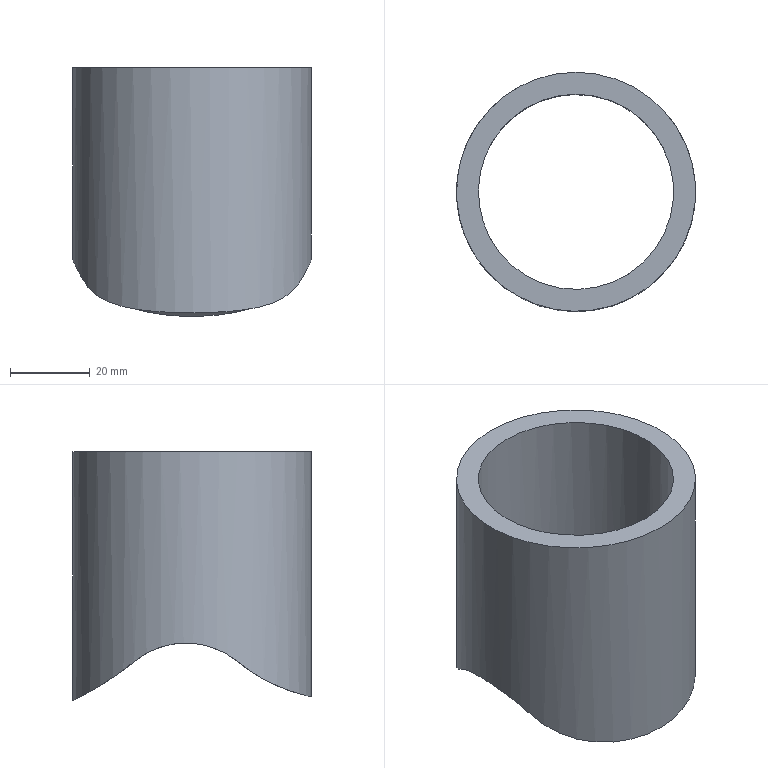Component | NX | CYLINDER | 1 solid | 7 faces | volume 52455 mm3 | cylinder 6 | plane 1 | commonest cylinder face diameters 40.874 x2 60 x1 49 x1 85.854 x1 148.319 x1